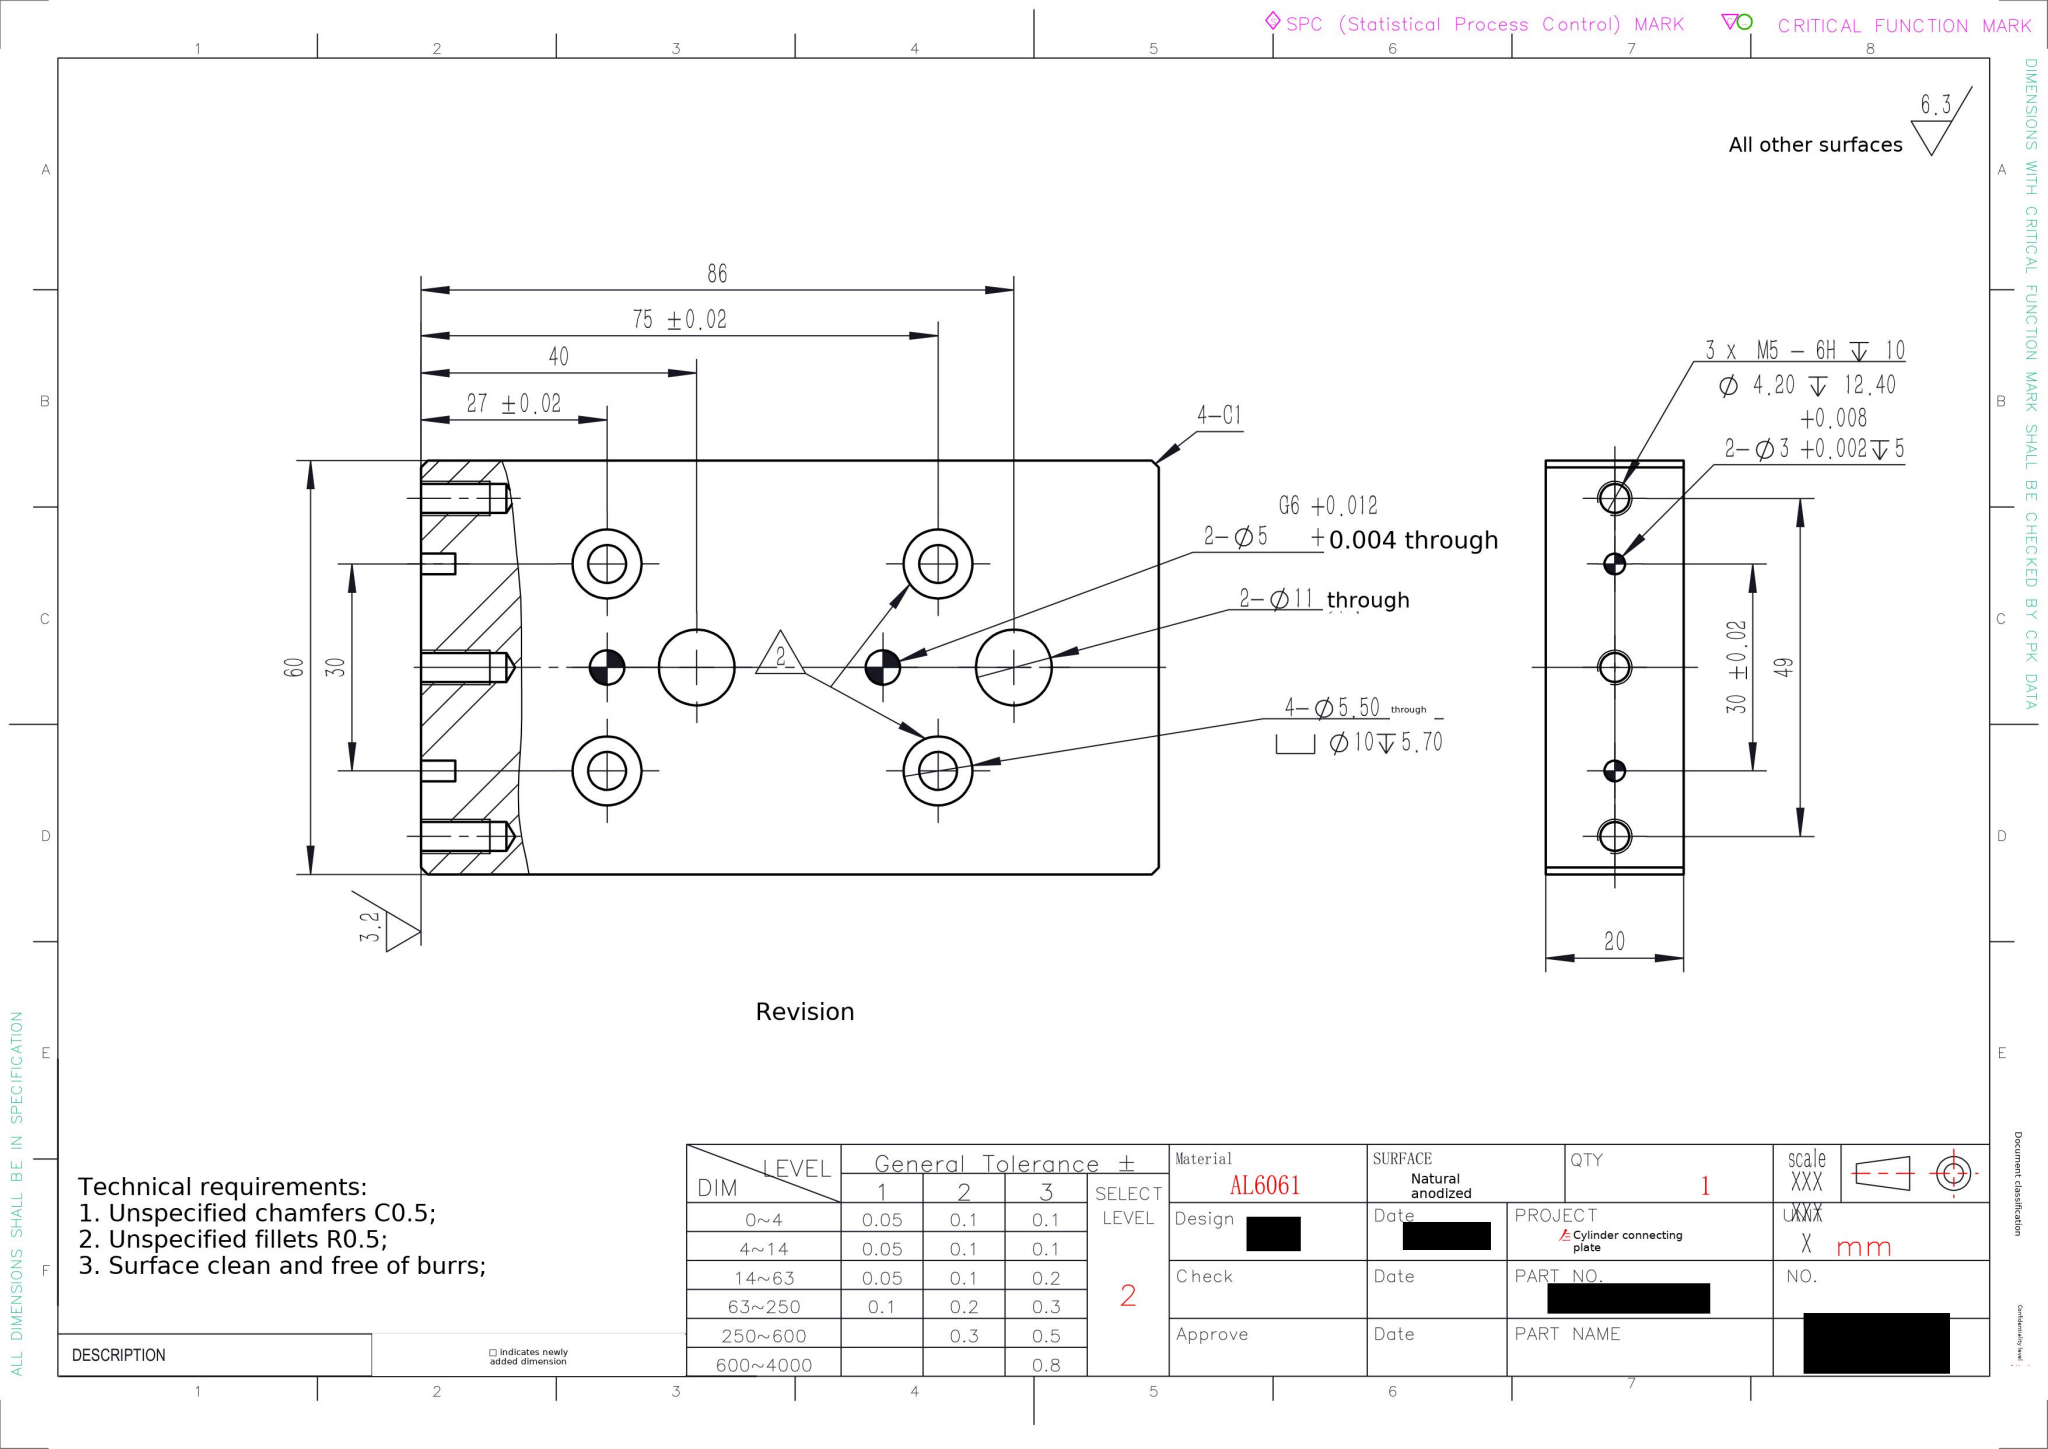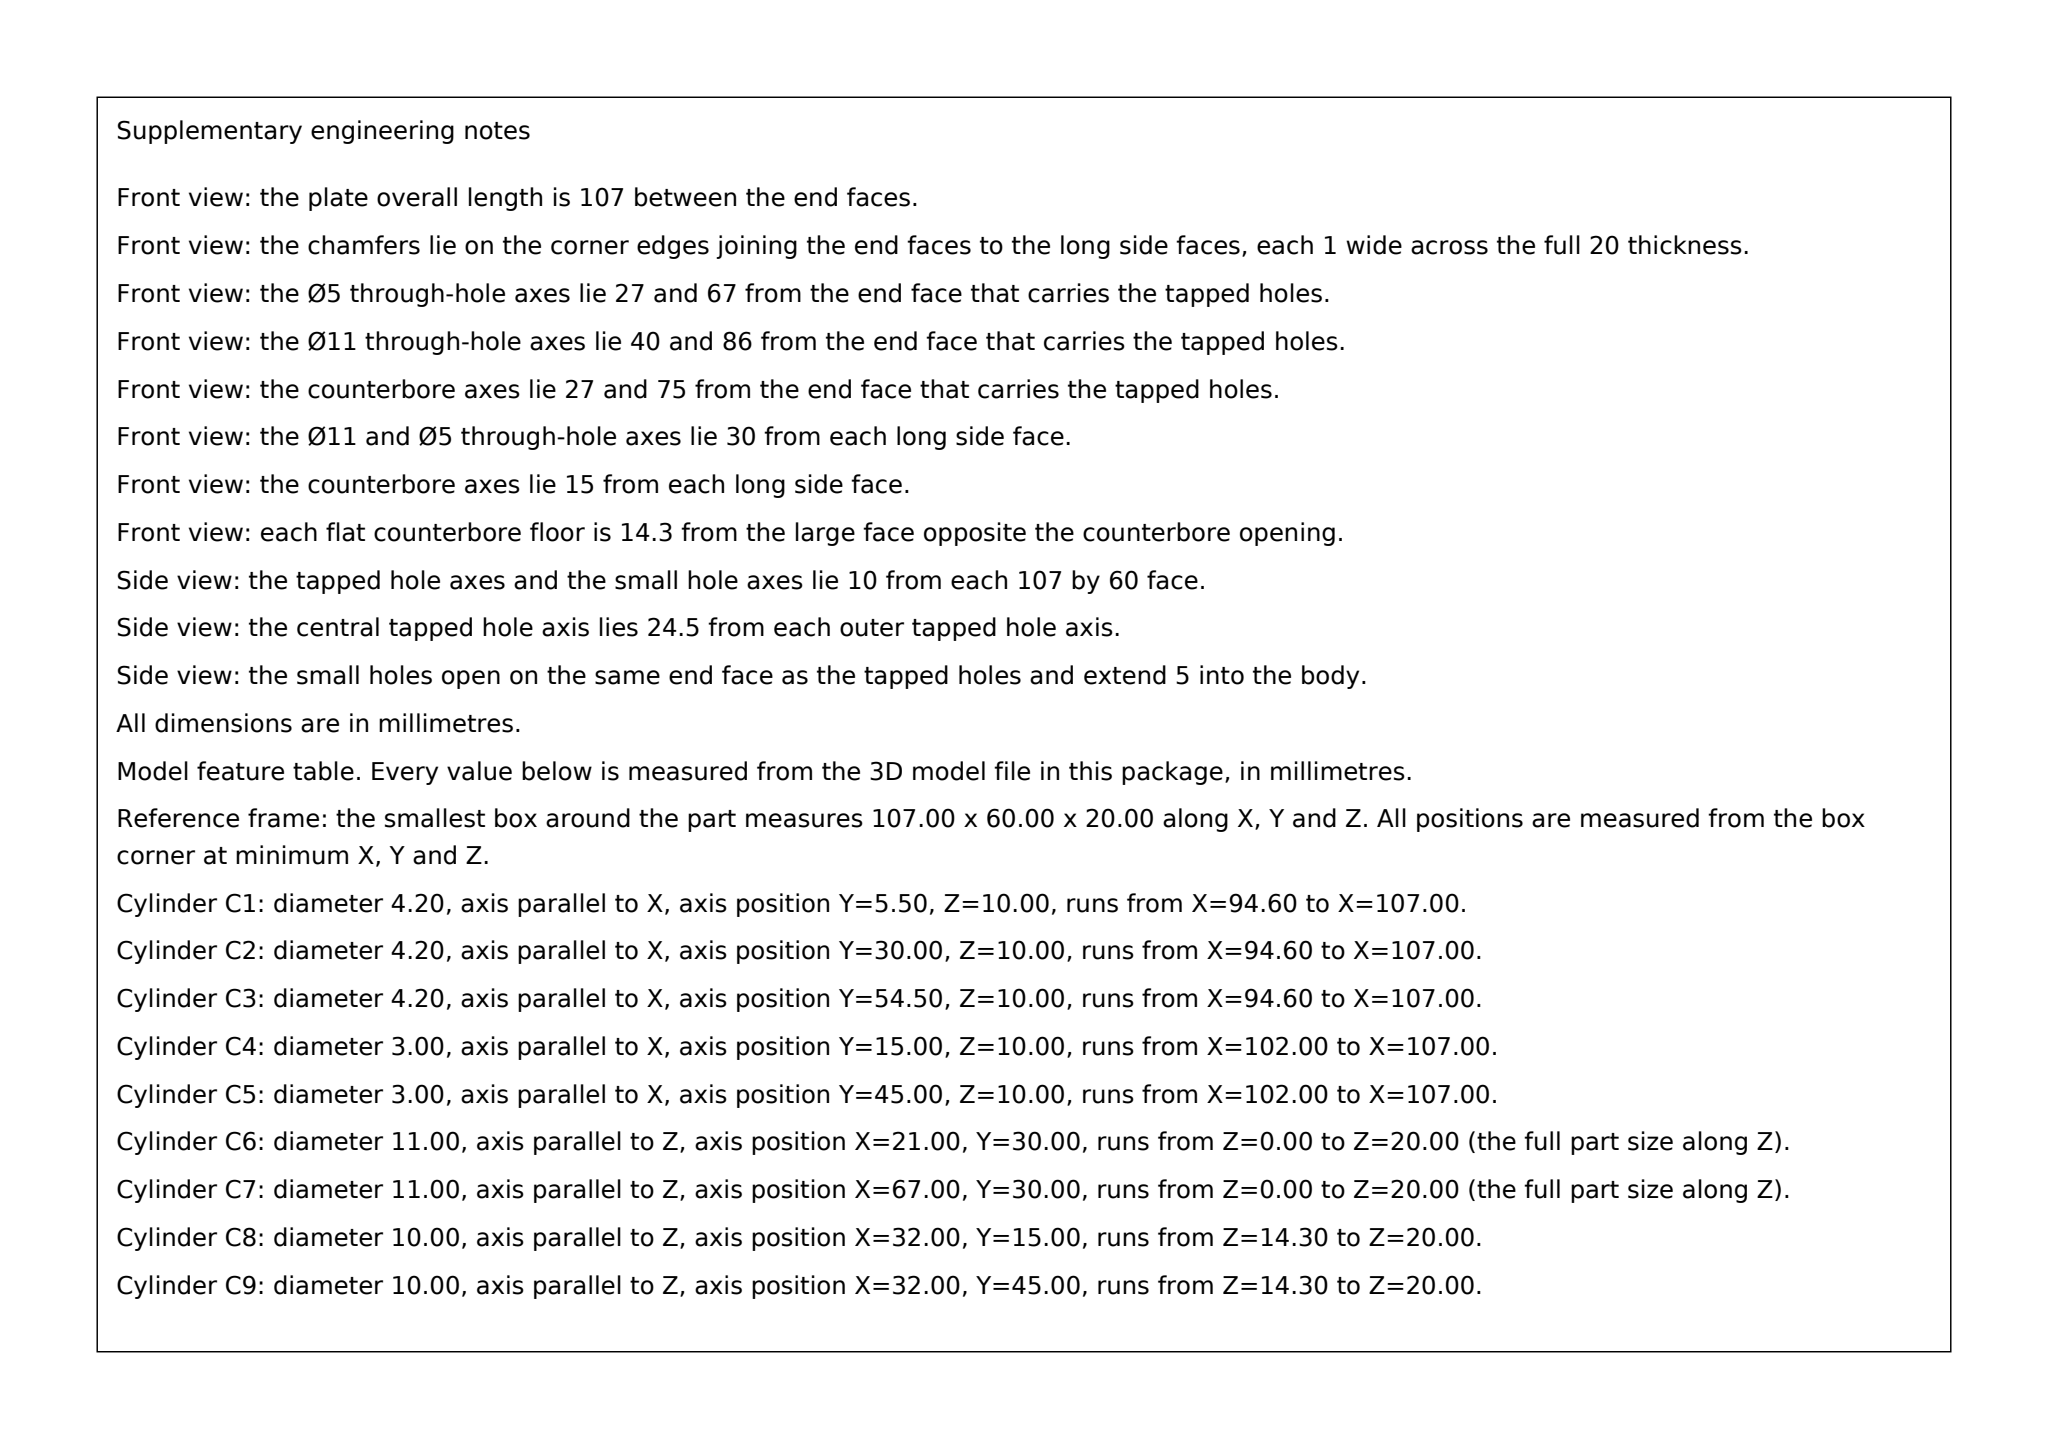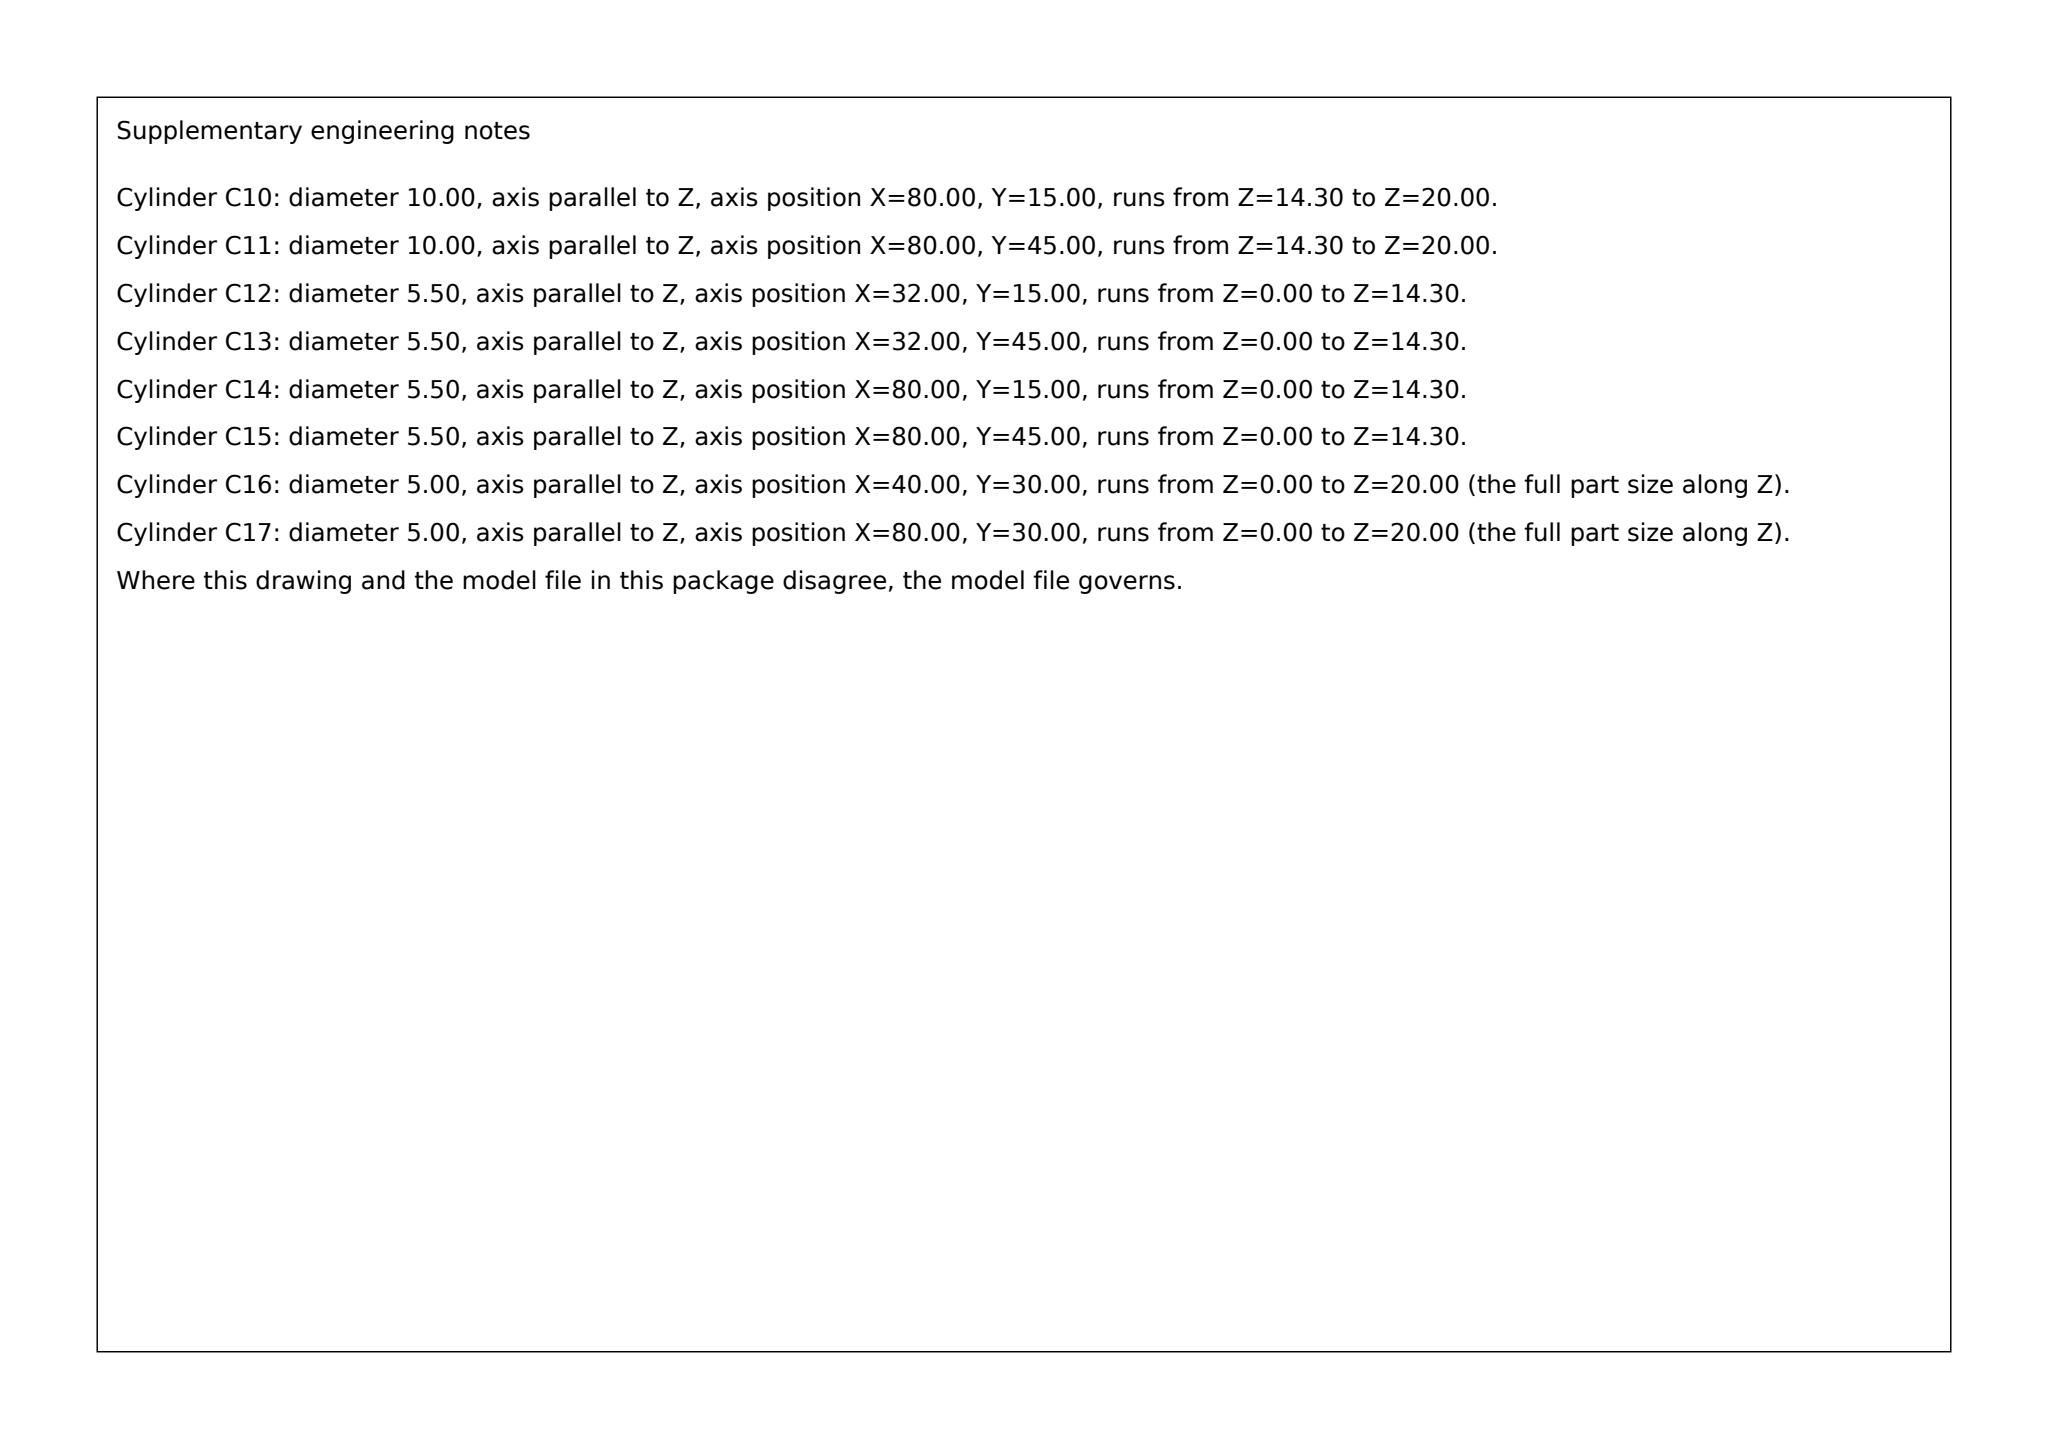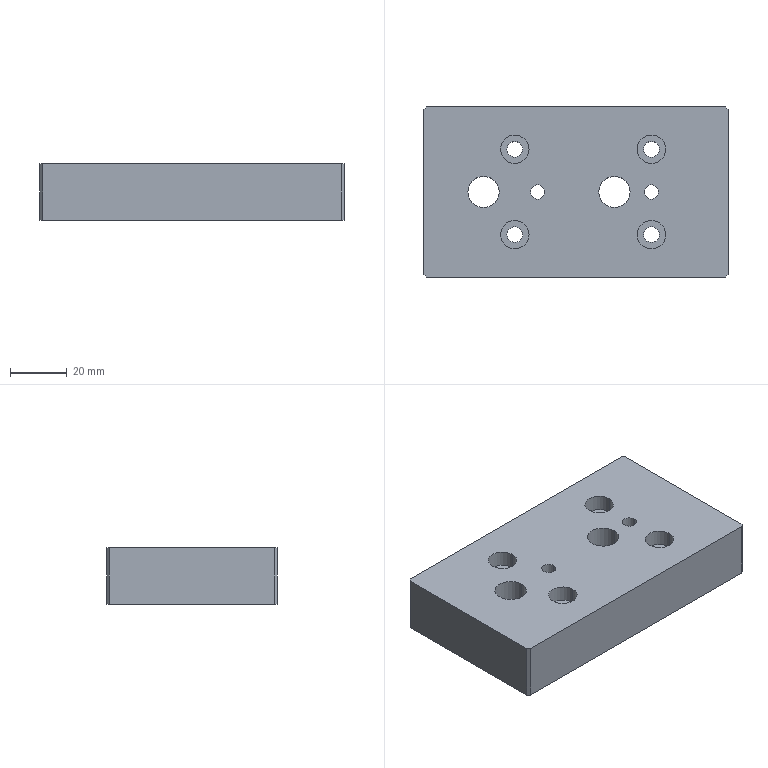Part | SolidWorks | mm | 1 solid | 56 faces | box 107 x 60 x 20 mm | volume 120020 mm3 | cylinder 34 | plane 16 | cone 6 | commonest cylinder face diameters 10 x8 5.5 x8 4.2 x6 3 x4 11 x4 5 x4
build123d program:
from build123d import *

# Parameters (mm, degrees)
SKETCH1_W                                         = 107
SKETCH1_H                                         = 60
BOSS_EXTRUDE1_DEPTH                               = 20
SKETCH3_R                                         = 2.5
CUT_EXTRUDE2_DEPTH                                = 65.516
HOLE_SIZE_ACCORDING_TO_HEXAGON_SOCKET_D           = 5.5
HOLE_SIZE_ACCORDING_TO_HEXAGON_SOCKET_CBORE_D     = 10
HOLE_SIZE_ACCORDING_TO_HEXAGON_SOCKET_CBORE_DEPTH = 5.7
SKETCH6_R                                         = 5.5
CUT_EXTRUDE3_DEPTH                                = 65.516
SKETCH7_R                                         = 1.5
CUT_EXTRUDE4_DEPTH                                = 5
M5_TAPPED_HOLE1_D                                 = 4.2
M5_TAPPED_HOLE1_DEPTH                             = 12.4
M5_TAPPED_HOLE1_TIP                               = 1.262
CHAMFER1_SIZE                                     = 1


with BuildPart() as part:
    # Sketch1 → Boss-Extrude1 (new body)
    with BuildSketch(Plane.XY):
        Rectangle(SKETCH1_W, SKETCH1_H)
    extrude(amount=BOSS_EXTRUDE1_DEPTH)

    # Sketch3 → Cut-Extrude2 (cut, through all)
    with BuildSketch(Plane.XY.offset(20)):
        with Locations((-13.5, 0)):
            Circle(SKETCH3_R)
        with Locations((26.5, 0)):
            Circle(SKETCH3_R)
    extrude(amount=-CUT_EXTRUDE2_DEPTH, mode=Mode.SUBTRACT)

    # Hole Size _ according to_ Hexagon Socket (through all)
    with Locations(Plane.XY.offset(20)):
        with Locations((-21.5, 15), (26.5, 15), (26.5, -15), (-21.5, -15)):
            CounterBoreHole(HOLE_SIZE_ACCORDING_TO_HEXAGON_SOCKET_D / 2, HOLE_SIZE_ACCORDING_TO_HEXAGON_SOCKET_CBORE_D / 2, HOLE_SIZE_ACCORDING_TO_HEXAGON_SOCKET_CBORE_DEPTH)

    # Sketch6 → Cut-Extrude3 (cut, through all)
    with BuildSketch(Plane.XY.offset(20)):
        with Locations((13.5, 0)):
            Circle(SKETCH6_R)
        with Locations((-32.5, 0)):
            Circle(SKETCH6_R)
    extrude(amount=-CUT_EXTRUDE3_DEPTH, mode=Mode.SUBTRACT)

    # Sketch7 → Cut-Extrude4 (cut)
    with BuildSketch(Plane(origin=(53.5, 0, 0), x_dir=(0, 0, -1), z_dir=(1, 0, 0))):
        with Locations(Location((-10, 15, 0), (0, 0, 90))):
            Circle(SKETCH7_R)
        with Locations(Location((-10, -15, 0), (0, 0, 270))):
            Circle(SKETCH7_R)
    extrude(amount=-CUT_EXTRUDE4_DEPTH, mode=Mode.SUBTRACT)

    # M5 Tapped Hole1
    with Locations(Plane(origin=(53.5, 0, 0), x_dir=(0, 0, -1), z_dir=(1, 0, 0))):
        with Locations((-10, 24.5), (-10, -24.5), (-10, 0)):
            Hole(M5_TAPPED_HOLE1_D / 2, depth=M5_TAPPED_HOLE1_DEPTH)
            with Locations((0, 0, -(M5_TAPPED_HOLE1_DEPTH + M5_TAPPED_HOLE1_TIP / 2))):  # 118° drill point
                Cone(0, M5_TAPPED_HOLE1_D / 2, M5_TAPPED_HOLE1_TIP, mode=Mode.SUBTRACT)

    # Chamfer1
    chamfer1_edges = [part.edges().sort_by_distance(p)[0] for p in [
        (53.5, -30, 10),
        (-53.5, -30, 10),
        (-53.5, 30, 10),
        (53.5, 30, 10),
    ]]
    chamfer(chamfer1_edges, length=CHAMFER1_SIZE)


solid = part.part